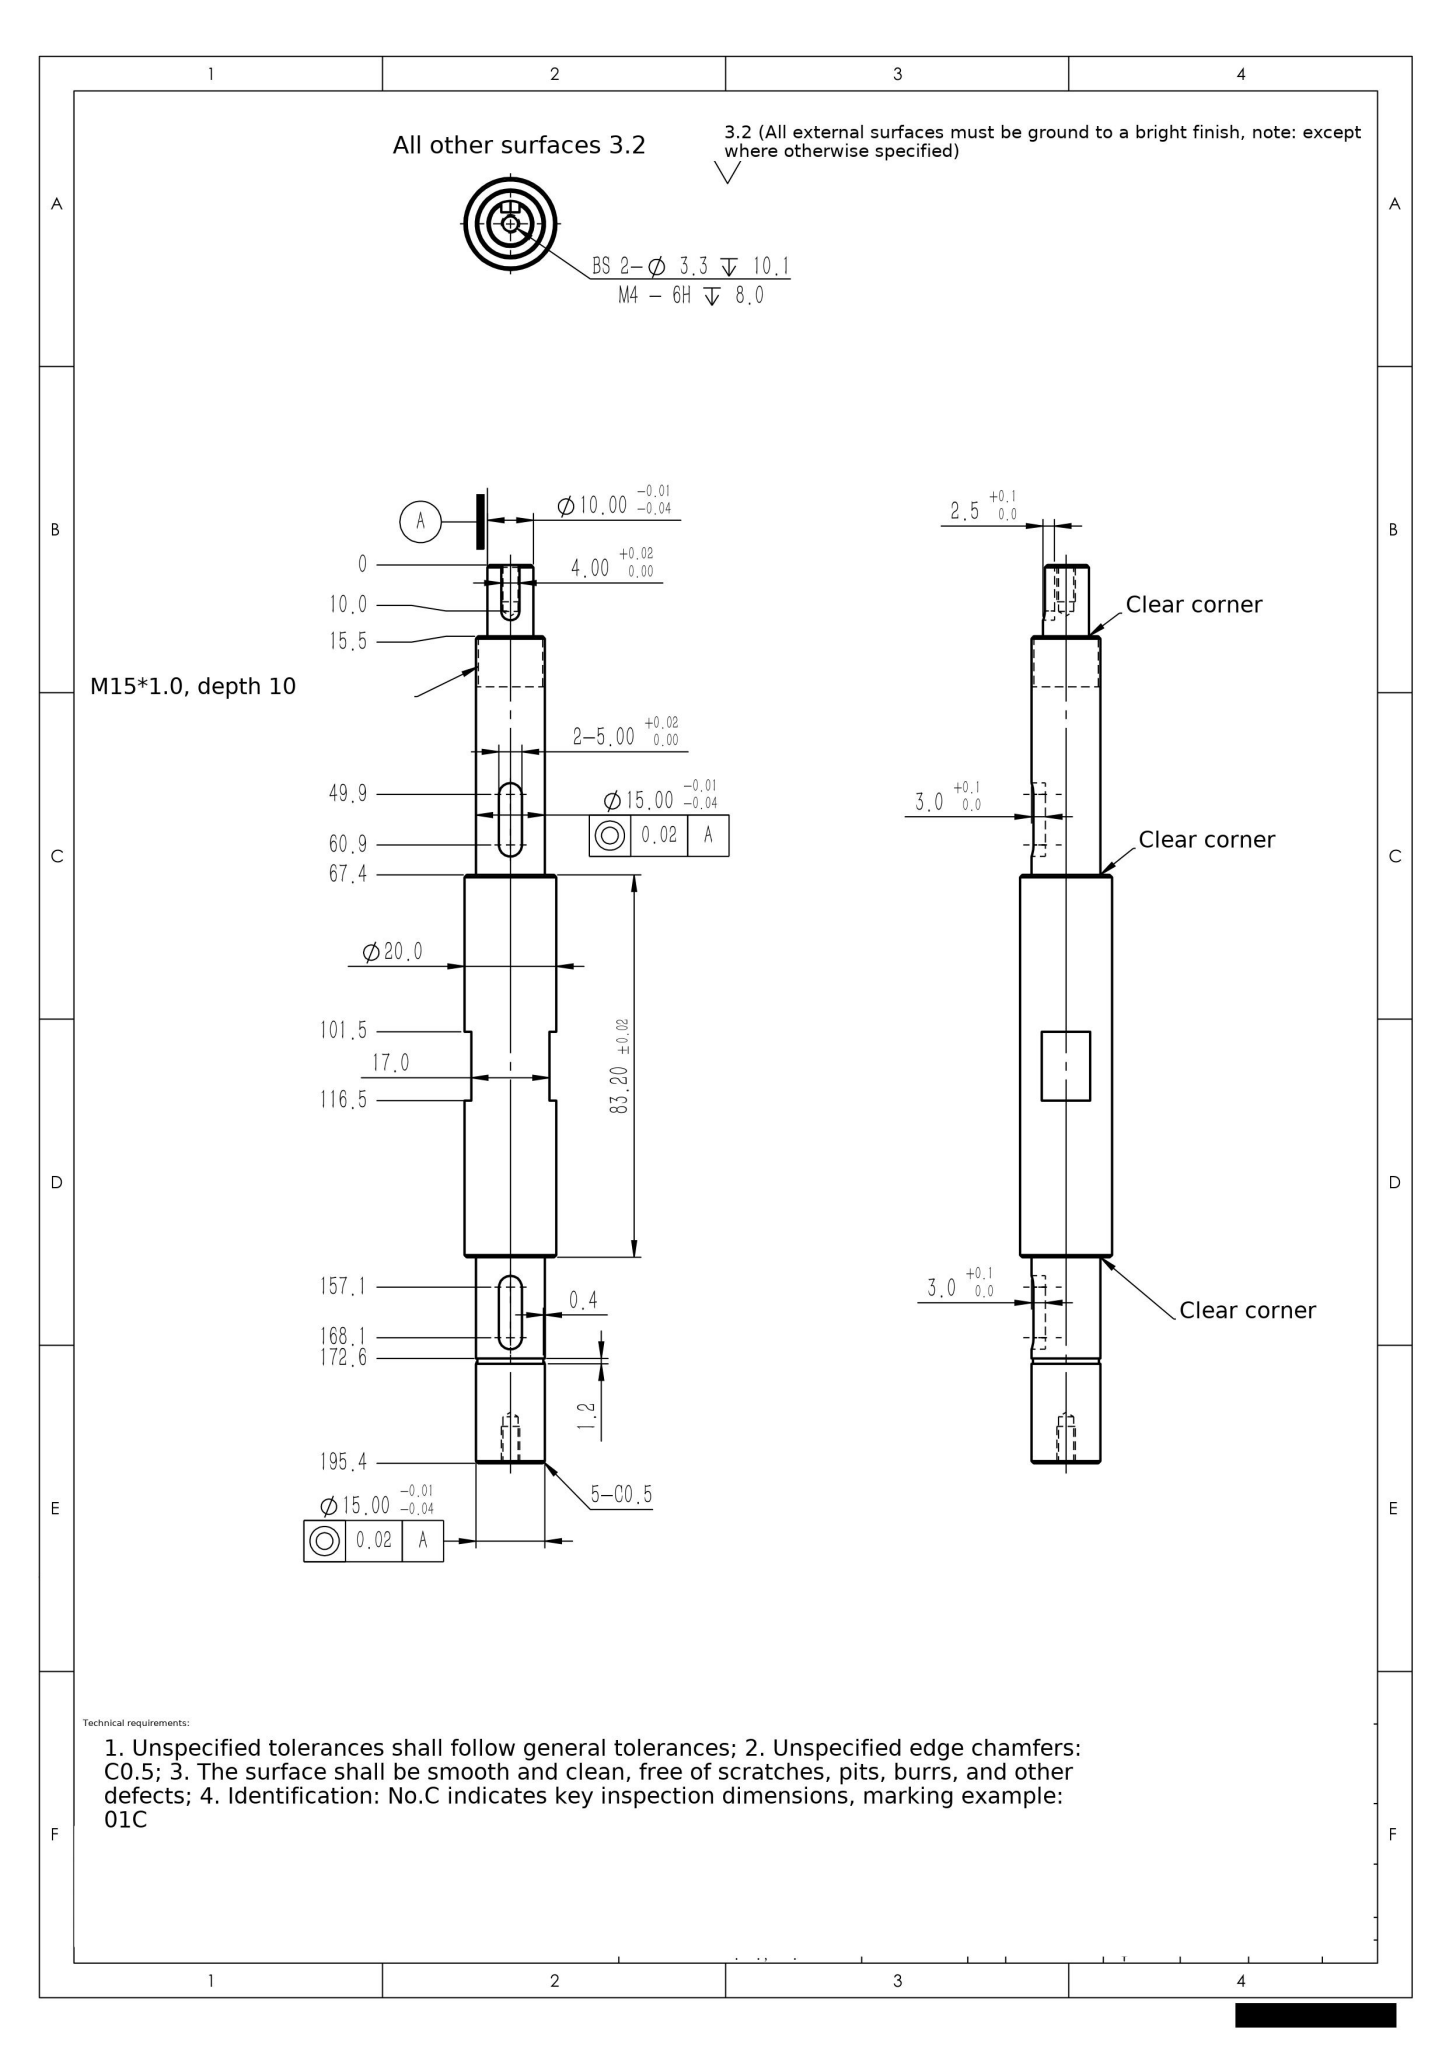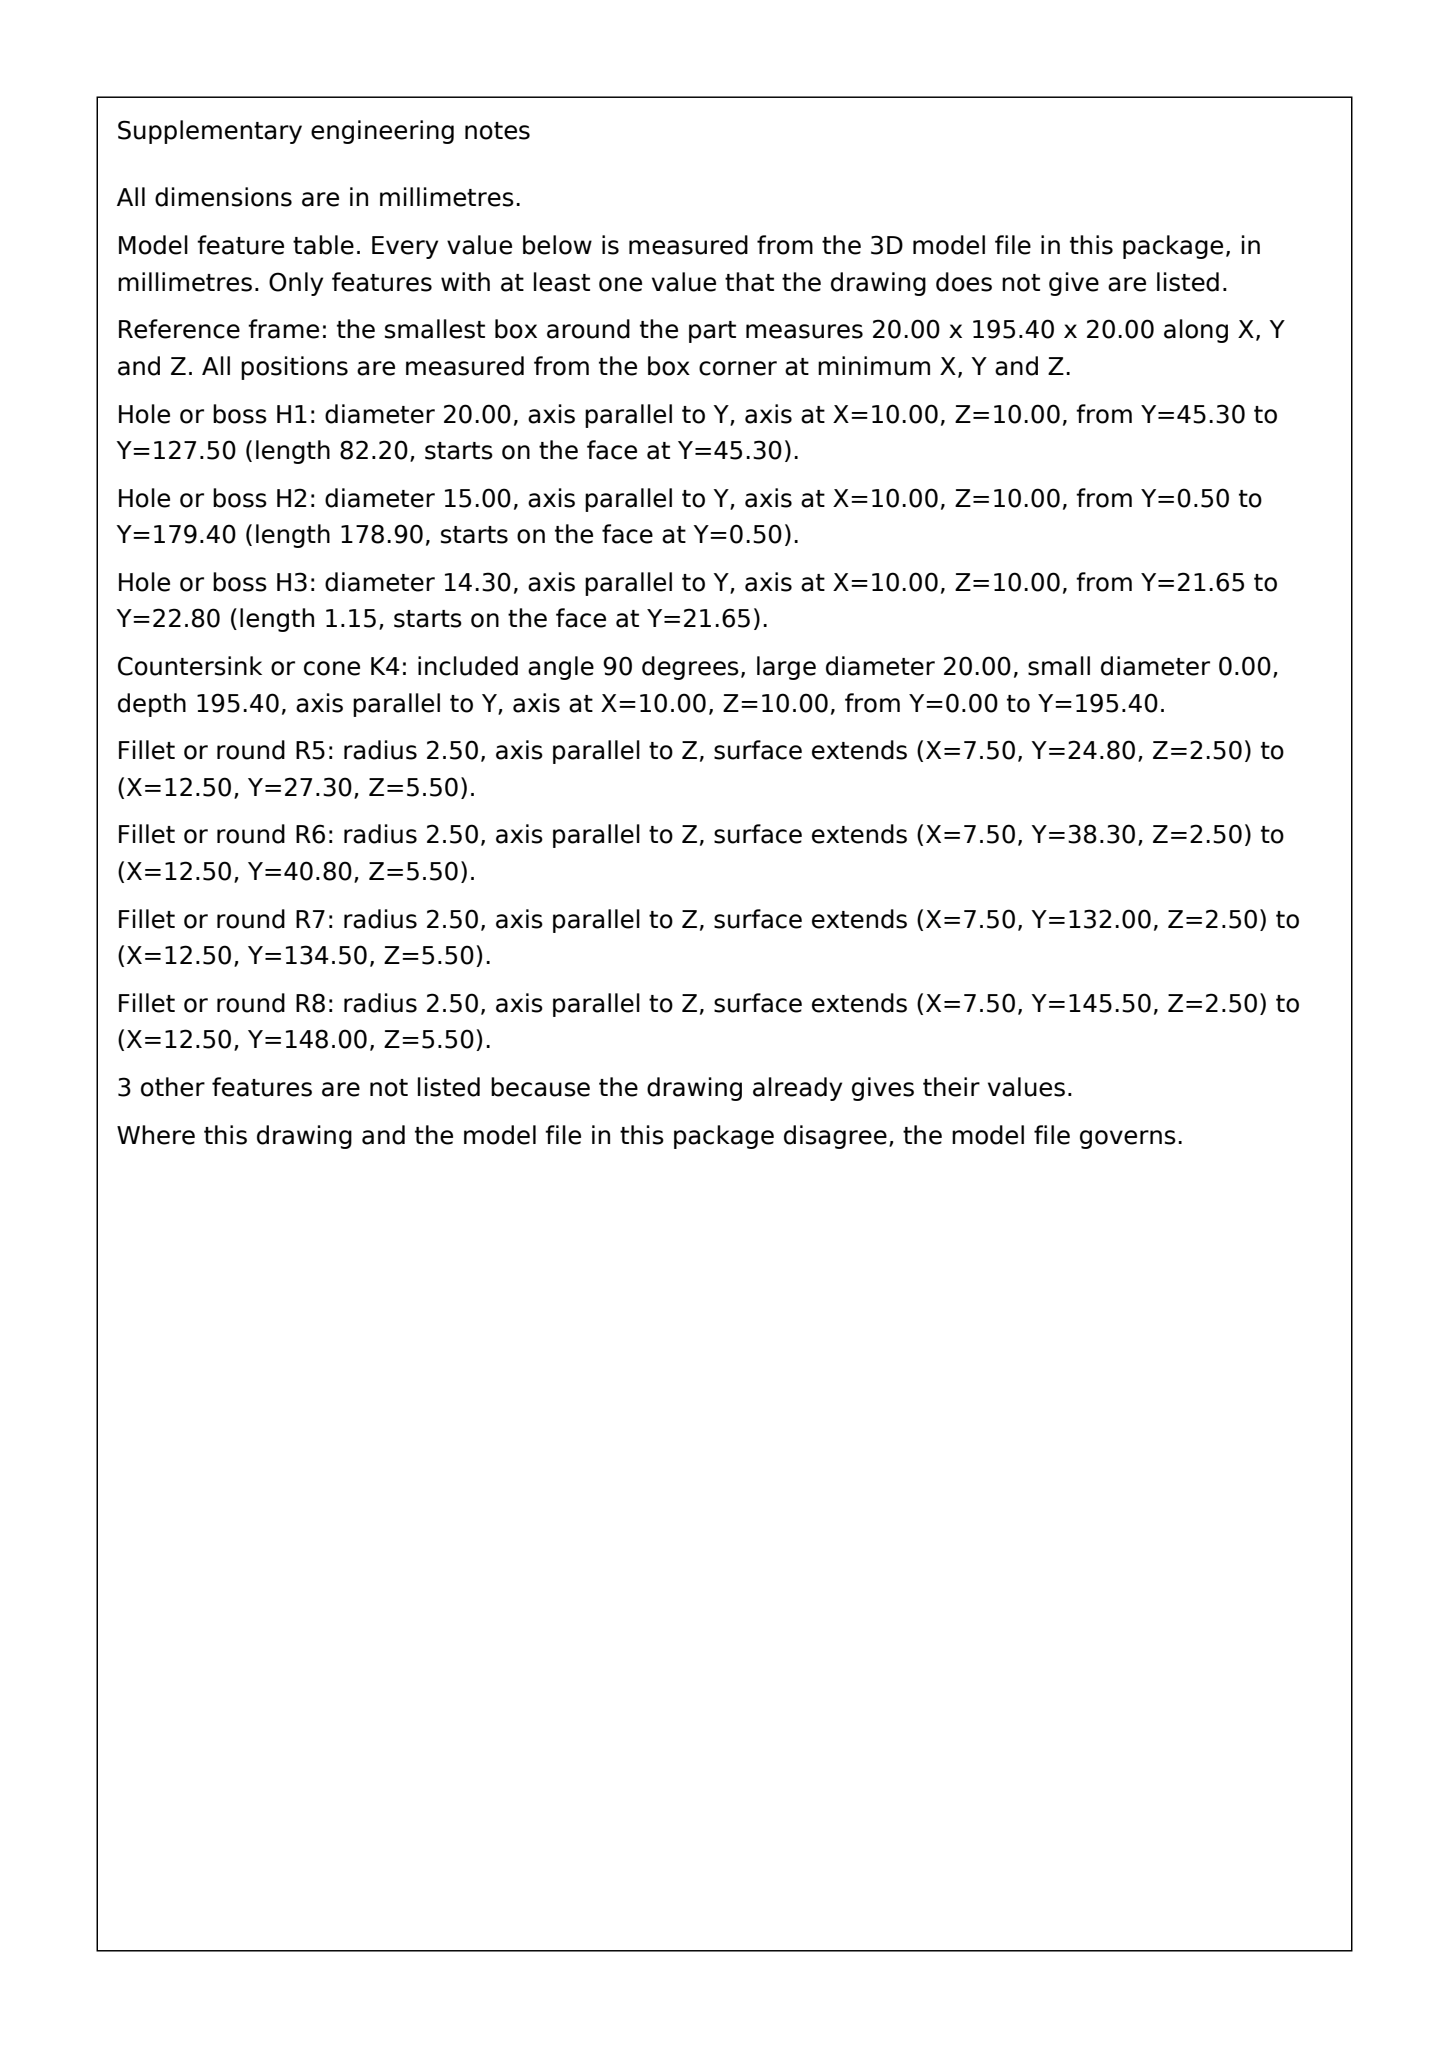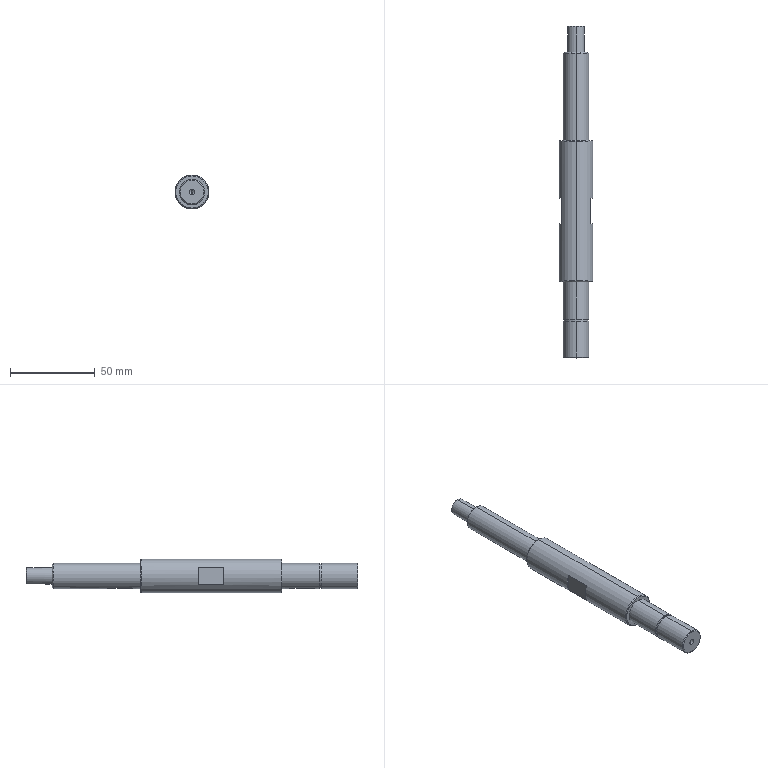Part | SolidWorks | mm | 1 solid | 57 faces | box 20 x 195.4 x 20 mm | volume 43358 mm3 | cylinder 22 | plane 22 | cone 13 | commonest cylinder face diameters 15 x6 3.3 x4 5 x4 14.3 x2 10 x2 20 x2 4 x2